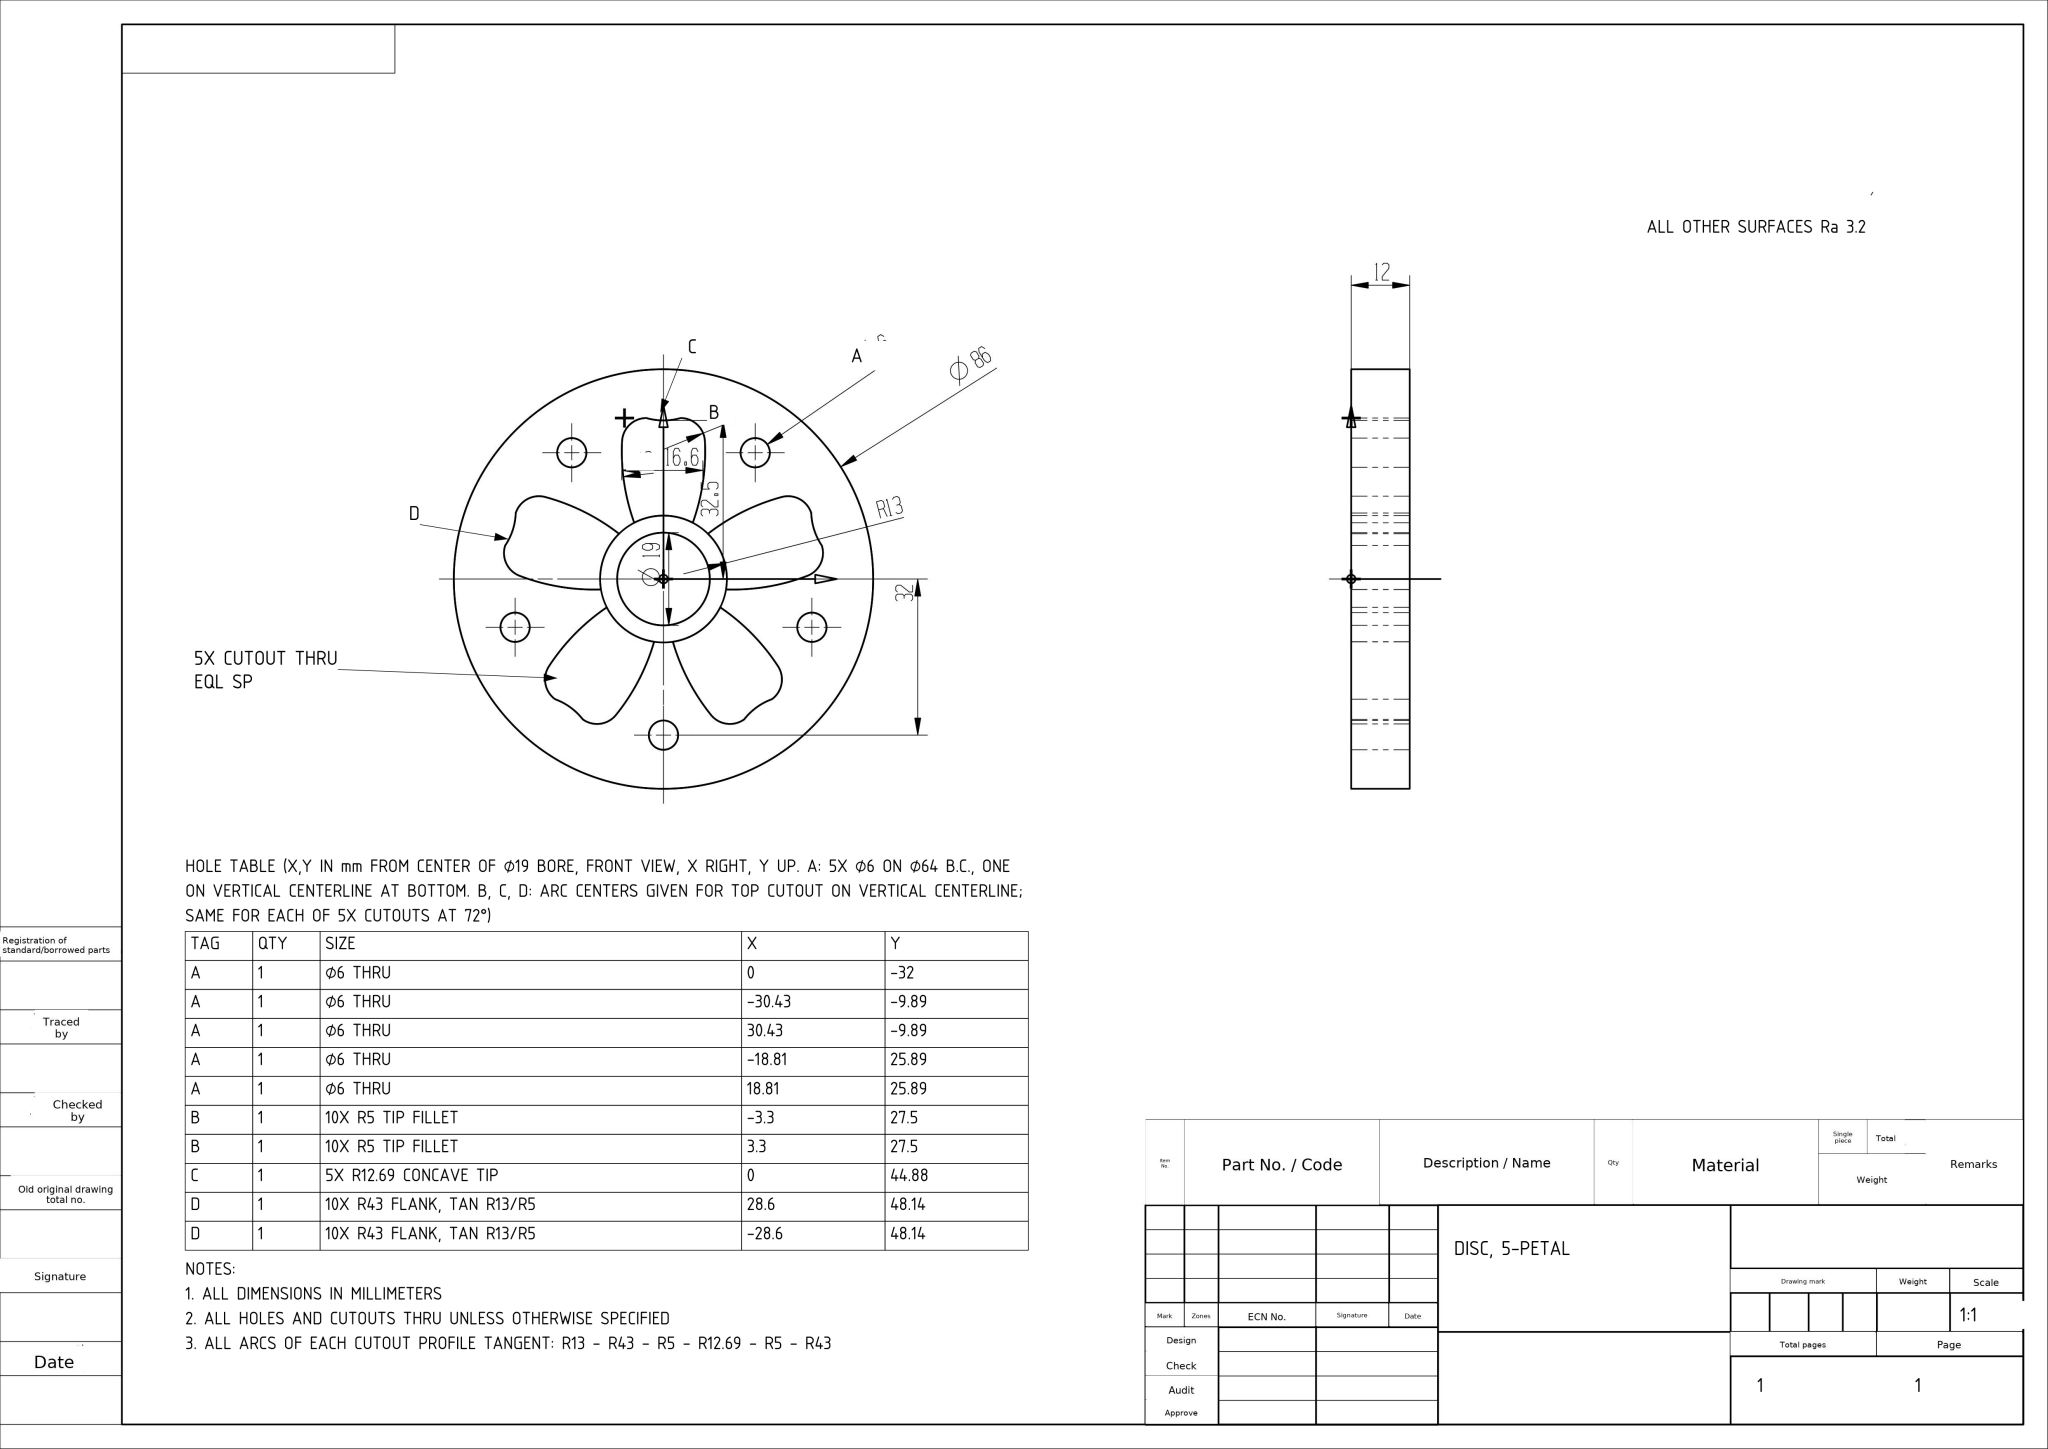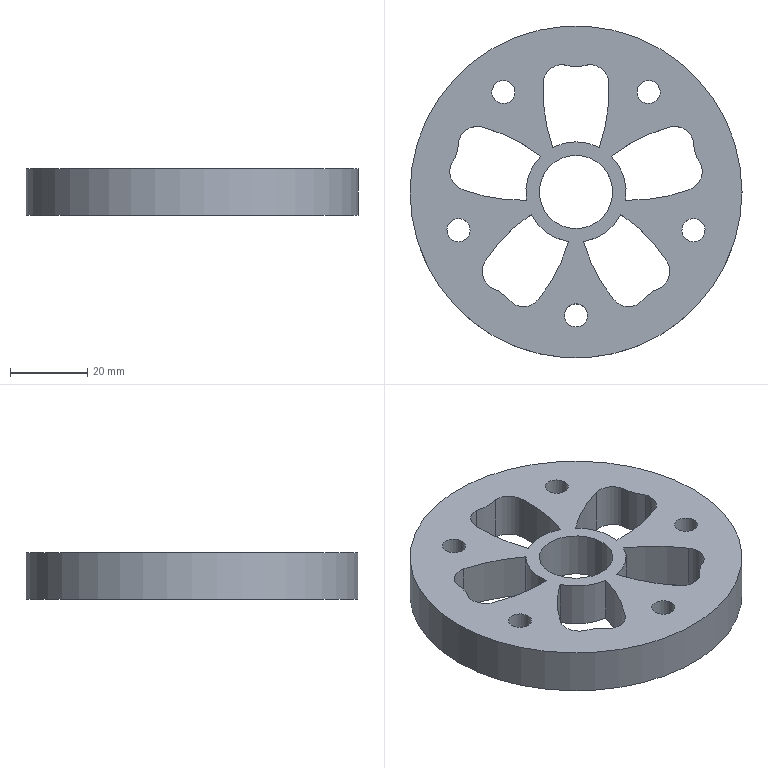Part | NX | mm | 1 solid | 39 faces | box 86 x 86 x 12 mm | volume 45582 mm3 | cylinder 37 | plane 2 | commonest cylinder face diameters 86 x11 10 x10 25.382 x5 6 x5 26 x5 19 x1